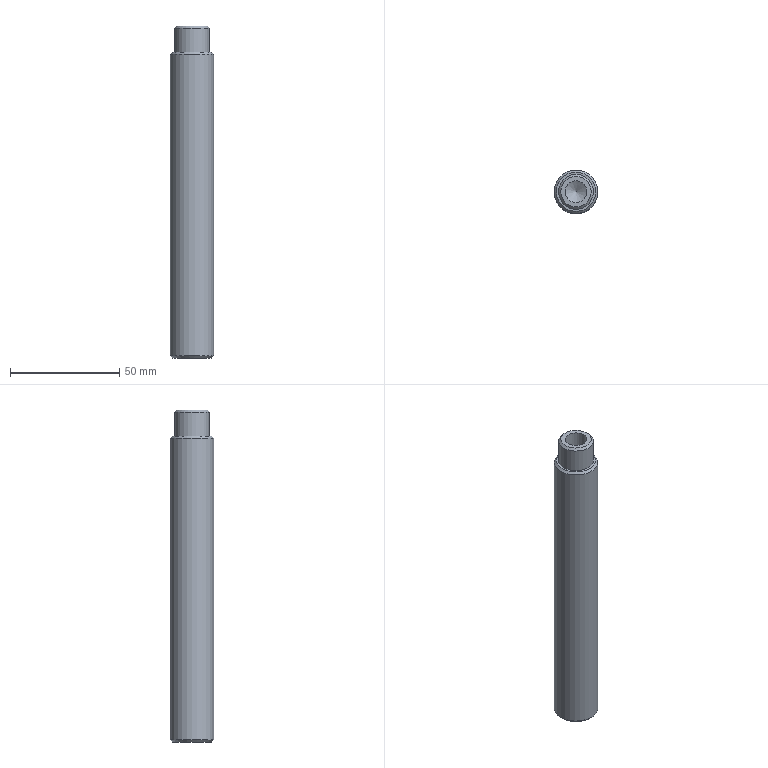Component | NX | STUD | 1 solid | 12 faces | box 20 x 20 x 152 mm | volume 43662 mm3 | cone 5 | cylinder 4 | plane 3 | commonest cylinder face diameters 20 x1 16 x1 6.8 x1 10 x1
STEP:
#1=CARTESIAN_POINT('',(0.,0.,0.));
#2=DIRECTION('',(0.,0.,1.));
#3=DIRECTION('',(1.,0.,0.));
#4=AXIS2_PLACEMENT_3D('',#1,#2,#3);
#5=CARTESIAN_POINT('',(-177.087,0.,160.));
#6=VERTEX_POINT('',#5);
#7=CARTESIAN_POINT('',(-186.087,0.,160.));
#8=DIRECTION('',(0.,0.,1.));
#9=DIRECTION('',(1.,0.,0.));
#10=AXIS2_PLACEMENT_3D('',#7,#8,#9);
#11=CIRCLE('',#10,9.);
#12=CARTESIAN_POINT('',(-186.087,0.,160.));
#13=DIRECTION('',(0.,0.,1.));
#14=DIRECTION('',(1.,0.,0.));
#15=AXIS2_PLACEMENT_3D('',#12,#13,#14);
#16=PLANE('',#15);
#17=CARTESIAN_POINT('',(0.,0.));
#18=DIRECTION('',(1.,0.));
#19=AXIS2_PLACEMENT_2D('',#17,#18);
#20=CIRCLE('',#19,9.);
#21=(GEOMETRIC_REPRESENTATION_CONTEXT(2)PARAMETRIC_REPRESENTATION_CONTEXT()REPRESENTATION_CONTEXT('',''));
#22=DEFINITIONAL_REPRESENTATION('',(#20),#21);
#23=PCURVE('',#16,#22);
#24=CARTESIAN_POINT('',(-186.087,0.,159.));
#25=DIRECTION('',(0.,0.,-1.));
#26=DIRECTION('',(-1.,0.,0.));
#27=AXIS2_PLACEMENT_3D('',#24,#25,#26);
#28=CONICAL_SURFACE('',#27,10.,0.7854);
#29=CARTESIAN_POINT('',(9.425,-1.));
#30=DIRECTION('',(-1.,0.));
#31=VECTOR('',#30,1.);
#32=LINE('',#29,#31);
#33=(GEOMETRIC_REPRESENTATION_CONTEXT(2)PARAMETRIC_REPRESENTATION_CONTEXT()REPRESENTATION_CONTEXT('',''));
#34=DEFINITIONAL_REPRESENTATION('',(#32),#33);
#35=PCURVE('',#28,#34);
#36=SURFACE_CURVE('',#11,(#23,#35),.PCURVE_S1.);
#37=EDGE_CURVE('',#6,#6,#36,.T.);
#38=ORIENTED_EDGE('',*,*,#37,.T.);
#39=EDGE_LOOP('',(#38));
#40=FACE_BOUND('',#39,.T.);
#41=CARTESIAN_POINT('',(-178.087,0.,160.));
#42=VERTEX_POINT('',#41);
#43=CARTESIAN_POINT('',(-186.087,0.,160.));
#44=DIRECTION('',(0.,0.,1.));
#45=DIRECTION('',(1.,0.,0.));
#46=AXIS2_PLACEMENT_3D('',#43,#44,#45);
#47=CIRCLE('',#46,8.);
#48=CARTESIAN_POINT('',(0.,0.));
#49=DIRECTION('',(1.,0.));
#50=AXIS2_PLACEMENT_2D('',#48,#49);
#51=CIRCLE('',#50,8.);
#52=(GEOMETRIC_REPRESENTATION_CONTEXT(2)PARAMETRIC_REPRESENTATION_CONTEXT()REPRESENTATION_CONTEXT('',''));
#53=DEFINITIONAL_REPRESENTATION('',(#51),#52);
#54=PCURVE('',#16,#53);
#55=CARTESIAN_POINT('',(-186.087,0.,172.));
#56=DIRECTION('',(0.,0.,-1.));
#57=DIRECTION('',(-1.,0.,0.));
#58=AXIS2_PLACEMENT_3D('',#55,#56,#57);
#59=CYLINDRICAL_SURFACE('',#58,8.);
#60=CARTESIAN_POINT('',(9.425,12.));
#61=DIRECTION('',(-1.,0.));
#62=VECTOR('',#61,1.);
#63=LINE('',#60,#62);
#64=(GEOMETRIC_REPRESENTATION_CONTEXT(2)PARAMETRIC_REPRESENTATION_CONTEXT()REPRESENTATION_CONTEXT('',''));
#65=DEFINITIONAL_REPRESENTATION('',(#63),#64);
#66=PCURVE('',#59,#65);
#67=SURFACE_CURVE('',#47,(#54,#66),.PCURVE_S1.);
#68=EDGE_CURVE('',#42,#42,#67,.T.);
#69=ORIENTED_EDGE('',*,*,#68,.F.);
#70=EDGE_LOOP('',(#69));
#71=FACE_BOUND('',#70,.T.);
#72=ADVANCED_FACE('',(#40,#71),#16,.T.);
#73=CARTESIAN_POINT('',(-195.087,0.,20.));
#74=VERTEX_POINT('',#73);
#75=CARTESIAN_POINT('',(-186.087,0.,20.));
#76=DIRECTION('',(0.,0.,-1.));
#77=DIRECTION('',(-1.,0.,0.));
#78=AXIS2_PLACEMENT_3D('',#75,#76,#77);
#79=CIRCLE('',#78,9.);
#80=CARTESIAN_POINT('',(-186.087,0.,20.));
#81=DIRECTION('',(0.,0.,-1.));
#82=DIRECTION('',(-1.,0.,0.));
#83=AXIS2_PLACEMENT_3D('',#80,#81,#82);
#84=PLANE('',#83);
#85=CARTESIAN_POINT('',(0.,0.));
#86=DIRECTION('',(1.,0.));
#87=AXIS2_PLACEMENT_2D('',#85,#86);
#88=CIRCLE('',#87,9.);
#89=(GEOMETRIC_REPRESENTATION_CONTEXT(2)PARAMETRIC_REPRESENTATION_CONTEXT()REPRESENTATION_CONTEXT('',''));
#90=DEFINITIONAL_REPRESENTATION('',(#88),#89);
#91=PCURVE('',#84,#90);
#92=CARTESIAN_POINT('',(-186.087,0.,21.));
#93=DIRECTION('',(0.,0.,1.));
#94=DIRECTION('',(1.,0.,0.));
#95=AXIS2_PLACEMENT_3D('',#92,#93,#94);
#96=CONICAL_SURFACE('',#95,10.,0.7854);
#97=CARTESIAN_POINT('',(9.425,-1.));
#98=DIRECTION('',(-1.,0.));
#99=VECTOR('',#98,1.);
#100=LINE('',#97,#99);
#101=(GEOMETRIC_REPRESENTATION_CONTEXT(2)PARAMETRIC_REPRESENTATION_CONTEXT()REPRESENTATION_CONTEXT('',''));
#102=DEFINITIONAL_REPRESENTATION('',(#100),#101);
#103=PCURVE('',#96,#102);
#104=SURFACE_CURVE('',#79,(#91,#103),.PCURVE_S1.);
#105=EDGE_CURVE('',#74,#74,#104,.T.);
#106=ORIENTED_EDGE('',*,*,#105,.T.);
#107=EDGE_LOOP('',(#106));
#108=FACE_BOUND('',#107,.T.);
#109=CARTESIAN_POINT('',(-182.687,0.,20.));
#110=VERTEX_POINT('',#109);
#111=CARTESIAN_POINT('',(-186.087,0.,20.));
#112=DIRECTION('',(0.,0.,1.));
#113=DIRECTION('',(1.,0.,0.));
#114=AXIS2_PLACEMENT_3D('',#111,#112,#113);
#115=CIRCLE('',#114,3.4);
#116=CARTESIAN_POINT('',(-3.4,0.));
#117=CARTESIAN_POINT('',(-3.4,5.889));
#118=CARTESIAN_POINT('',(1.7,2.944));
#119=CARTESIAN_POINT('',(6.8,0.));
#120=CARTESIAN_POINT('',(1.7,-2.944));
#121=CARTESIAN_POINT('',(-3.4,-5.889));
#122=CARTESIAN_POINT('',(-3.4,0.));
#123=(BOUNDED_CURVE()B_SPLINE_CURVE(2,(#116,#117,#118,#119,#120,#121,#122),.UNSPECIFIED.,.T.,.F.)B_SPLINE_CURVE_WITH_KNOTS((1,2,2,2,2,1),(-2.094,0.,2.094,4.189,6.283,8.378),.UNSPECIFIED.)CURVE()GEOMETRIC_REPRESENTATION_ITEM()RATIONAL_B_SPLINE_CURVE((1.,0.5,1.,0.5,1.,0.5,1.))REPRESENTATION_ITEM(''));
#124=(GEOMETRIC_REPRESENTATION_CONTEXT(2)PARAMETRIC_REPRESENTATION_CONTEXT()REPRESENTATION_CONTEXT('',''));
#125=DEFINITIONAL_REPRESENTATION('',(#123),#124);
#126=PCURVE('',#84,#125);
#127=CARTESIAN_POINT('',(-186.087,0.,20.));
#128=DIRECTION('',(0.,0.,1.));
#129=DIRECTION('',(1.,0.,0.));
#130=AXIS2_PLACEMENT_3D('',#127,#128,#129);
#131=CYLINDRICAL_SURFACE('',#130,3.4);
#132=CARTESIAN_POINT('',(0.,0.));
#133=DIRECTION('',(1.,0.));
#134=VECTOR('',#133,1.);
#135=LINE('',#132,#134);
#136=(GEOMETRIC_REPRESENTATION_CONTEXT(2)PARAMETRIC_REPRESENTATION_CONTEXT()REPRESENTATION_CONTEXT('',''));
#137=DEFINITIONAL_REPRESENTATION('',(#135),#136);
#138=PCURVE('',#131,#137);
#139=SURFACE_CURVE('',#115,(#126,#138),.PCURVE_S1.);
#140=EDGE_CURVE('',#110,#110,#139,.T.);
#141=ORIENTED_EDGE('',*,*,#140,.T.);
#142=EDGE_LOOP('',(#141));
#143=FACE_BOUND('',#142,.T.);
#144=ADVANCED_FACE('',(#108,#143),#84,.T.);
#145=CARTESIAN_POINT('',(-176.087,0.,159.));
#146=VERTEX_POINT('',#145);
#147=CARTESIAN_POINT('',(-186.087,0.,159.));
#148=DIRECTION('',(0.,0.,-1.));
#149=DIRECTION('',(1.,0.,0.));
#150=AXIS2_PLACEMENT_3D('',#147,#148,#149);
#151=CIRCLE('',#150,10.);
#152=CARTESIAN_POINT('',(-186.087,0.,20.));
#153=DIRECTION('',(0.,0.,1.));
#154=DIRECTION('',(1.,0.,0.));
#155=AXIS2_PLACEMENT_3D('',#152,#153,#154);
#156=CYLINDRICAL_SURFACE('',#155,10.);
#157=CARTESIAN_POINT('',(6.283,139.));
#158=DIRECTION('',(-1.,0.));
#159=VECTOR('',#158,1.);
#160=LINE('',#157,#159);
#161=(GEOMETRIC_REPRESENTATION_CONTEXT(2)PARAMETRIC_REPRESENTATION_CONTEXT()REPRESENTATION_CONTEXT('',''));
#162=DEFINITIONAL_REPRESENTATION('',(#160),#161);
#163=PCURVE('',#156,#162);
#164=CARTESIAN_POINT('',(3.142,0.));
#165=DIRECTION('',(1.,0.));
#166=VECTOR('',#165,1.);
#167=LINE('',#164,#166);
#168=(GEOMETRIC_REPRESENTATION_CONTEXT(2)PARAMETRIC_REPRESENTATION_CONTEXT()REPRESENTATION_CONTEXT('',''));
#169=DEFINITIONAL_REPRESENTATION('',(#167),#168);
#170=PCURVE('',#28,#169);
#171=SURFACE_CURVE('',#151,(#163,#170),.PCURVE_S1.);
#172=EDGE_CURVE('',#146,#146,#171,.T.);
#173=ORIENTED_EDGE('',*,*,#172,.T.);
#174=CARTESIAN_POINT('',(-176.087,0.,21.));
#175=VERTEX_POINT('',#174);
#176=CARTESIAN_POINT('',(-176.087,0.,21.));
#177=CARTESIAN_POINT('',(-176.087,0.,159.));
#178=B_SPLINE_CURVE_WITH_KNOTS('',1,(#176,#177),.UNSPECIFIED.,.F.,.F.,(2,2),(1.,139.),.PIECEWISE_BEZIER_KNOTS.);
#179=CARTESIAN_POINT('',(0.,0.));
#180=DIRECTION('',(0.,1.));
#181=VECTOR('',#180,1.);
#182=LINE('',#179,#181);
#183=(GEOMETRIC_REPRESENTATION_CONTEXT(2)PARAMETRIC_REPRESENTATION_CONTEXT()REPRESENTATION_CONTEXT('',''));
#184=DEFINITIONAL_REPRESENTATION('',(#182),#183);
#185=PCURVE('',#156,#184);
#186=CARTESIAN_POINT('',(6.283,0.));
#187=DIRECTION('',(0.,1.));
#188=VECTOR('',#187,1.);
#189=LINE('',#186,#188);
#190=(GEOMETRIC_REPRESENTATION_CONTEXT(2)PARAMETRIC_REPRESENTATION_CONTEXT()REPRESENTATION_CONTEXT('',''));
#191=DEFINITIONAL_REPRESENTATION('',(#189),#190);
#192=PCURVE('',#156,#191);
#193=SEAM_CURVE('',#178,(#185,#192),.PCURVE_S1.);
#194=EDGE_CURVE('',#175,#146,#193,.T.);
#195=ORIENTED_EDGE('',*,*,#194,.F.);
#196=CARTESIAN_POINT('',(-196.087,0.,21.));
#197=VERTEX_POINT('',#196);
#198=CARTESIAN_POINT('',(-186.087,0.,21.));
#199=DIRECTION('',(0.,0.,1.));
#200=DIRECTION('',(-1.,0.,0.));
#201=AXIS2_PLACEMENT_3D('',#198,#199,#200);
#202=CIRCLE('',#201,10.);
#203=CARTESIAN_POINT('',(-3.142,1.));
#204=DIRECTION('',(1.,0.));
#205=VECTOR('',#204,1.);
#206=LINE('',#203,#205);
#207=(GEOMETRIC_REPRESENTATION_CONTEXT(2)PARAMETRIC_REPRESENTATION_CONTEXT()REPRESENTATION_CONTEXT('',''));
#208=DEFINITIONAL_REPRESENTATION('',(#206),#207);
#209=PCURVE('',#156,#208);
#210=CARTESIAN_POINT('',(3.142,0.));
#211=DIRECTION('',(1.,0.));
#212=VECTOR('',#211,1.);
#213=LINE('',#210,#212);
#214=(GEOMETRIC_REPRESENTATION_CONTEXT(2)PARAMETRIC_REPRESENTATION_CONTEXT()REPRESENTATION_CONTEXT('',''));
#215=DEFINITIONAL_REPRESENTATION('',(#213),#214);
#216=PCURVE('',#96,#215);
#217=SURFACE_CURVE('',#202,(#209,#216),.PCURVE_S1.);
#218=EDGE_CURVE('',#175,#197,#217,.T.);
#219=ORIENTED_EDGE('',*,*,#218,.T.);
#220=CARTESIAN_POINT('',(-186.087,0.,21.));
#221=DIRECTION('',(0.,0.,1.));
#222=DIRECTION('',(-1.,0.,0.));
#223=AXIS2_PLACEMENT_3D('',#220,#221,#222);
#224=CIRCLE('',#223,10.);
#225=CARTESIAN_POINT('',(3.142,1.));
#226=DIRECTION('',(1.,0.));
#227=VECTOR('',#226,1.);
#228=LINE('',#225,#227);
#229=(GEOMETRIC_REPRESENTATION_CONTEXT(2)PARAMETRIC_REPRESENTATION_CONTEXT()REPRESENTATION_CONTEXT('',''));
#230=DEFINITIONAL_REPRESENTATION('',(#228),#229);
#231=PCURVE('',#156,#230);
#232=CARTESIAN_POINT('',(3.142,0.));
#233=DIRECTION('',(1.,0.));
#234=VECTOR('',#233,1.);
#235=LINE('',#232,#234);
#236=(GEOMETRIC_REPRESENTATION_CONTEXT(2)PARAMETRIC_REPRESENTATION_CONTEXT()REPRESENTATION_CONTEXT('',''));
#237=DEFINITIONAL_REPRESENTATION('',(#235),#236);
#238=PCURVE('',#96,#237);
#239=SURFACE_CURVE('',#224,(#231,#238),.PCURVE_S1.);
#240=EDGE_CURVE('',#197,#175,#239,.T.);
#241=ORIENTED_EDGE('',*,*,#240,.T.);
#242=ORIENTED_EDGE('',*,*,#194,.T.);
#243=EDGE_LOOP('',(#173,#195,#219,#241,#242));
#244=FACE_BOUND('',#243,.T.);
#245=ADVANCED_FACE('',(#244),#156,.T.);
#246=CARTESIAN_POINT('',(-178.087,0.,171.));
#247=VERTEX_POINT('',#246);
#248=CARTESIAN_POINT('',(-186.087,0.,171.));
#249=DIRECTION('',(0.,0.,-1.));
#250=DIRECTION('',(1.,0.,0.));
#251=AXIS2_PLACEMENT_3D('',#248,#249,#250);
#252=CIRCLE('',#251,8.);
#253=CARTESIAN_POINT('',(3.142,1.));
#254=DIRECTION('',(1.,0.));
#255=VECTOR('',#254,1.);
#256=LINE('',#253,#255);
#257=(GEOMETRIC_REPRESENTATION_CONTEXT(2)PARAMETRIC_REPRESENTATION_CONTEXT()REPRESENTATION_CONTEXT('',''));
#258=DEFINITIONAL_REPRESENTATION('',(#256),#257);
#259=PCURVE('',#59,#258);
#260=CARTESIAN_POINT('',(-186.087,0.,172.));
#261=DIRECTION('',(0.,0.,-1.));
#262=DIRECTION('',(-1.,0.,0.));
#263=AXIS2_PLACEMENT_3D('',#260,#261,#262);
#264=CONICAL_SURFACE('',#263,7.,0.7854);
#265=CARTESIAN_POINT('',(3.142,1.));
#266=DIRECTION('',(1.,0.));
#267=VECTOR('',#266,1.);
#268=LINE('',#265,#267);
#269=(GEOMETRIC_REPRESENTATION_CONTEXT(2)PARAMETRIC_REPRESENTATION_CONTEXT()REPRESENTATION_CONTEXT('',''));
#270=DEFINITIONAL_REPRESENTATION('',(#268),#269);
#271=PCURVE('',#264,#270);
#272=SURFACE_CURVE('',#252,(#259,#271),.PCURVE_S1.);
#273=EDGE_CURVE('',#247,#247,#272,.T.);
#274=ORIENTED_EDGE('',*,*,#273,.T.);
#275=CARTESIAN_POINT('',(-178.087,0.,171.));
#276=CARTESIAN_POINT('',(-178.087,0.,160.));
#277=B_SPLINE_CURVE_WITH_KNOTS('',1,(#275,#276),.UNSPECIFIED.,.F.,.F.,(2,2),(1.,12.),.PIECEWISE_BEZIER_KNOTS.);
#278=CARTESIAN_POINT('',(9.425,0.));
#279=DIRECTION('',(0.,1.));
#280=VECTOR('',#279,1.);
#281=LINE('',#278,#280);
#282=(GEOMETRIC_REPRESENTATION_CONTEXT(2)PARAMETRIC_REPRESENTATION_CONTEXT()REPRESENTATION_CONTEXT('',''));
#283=DEFINITIONAL_REPRESENTATION('',(#281),#282);
#284=PCURVE('',#59,#283);
#285=CARTESIAN_POINT('',(3.142,0.));
#286=DIRECTION('',(0.,1.));
#287=VECTOR('',#286,1.);
#288=LINE('',#285,#287);
#289=(GEOMETRIC_REPRESENTATION_CONTEXT(2)PARAMETRIC_REPRESENTATION_CONTEXT()REPRESENTATION_CONTEXT('',''));
#290=DEFINITIONAL_REPRESENTATION('',(#288),#289);
#291=PCURVE('',#59,#290);
#292=SEAM_CURVE('',#277,(#284,#291),.PCURVE_S1.);
#293=EDGE_CURVE('',#247,#42,#292,.T.);
#294=ORIENTED_EDGE('',*,*,#293,.T.);
#295=ORIENTED_EDGE('',*,*,#68,.T.);
#296=ORIENTED_EDGE('',*,*,#293,.F.);
#297=EDGE_LOOP('',(#274,#294,#295,#296));
#298=FACE_BOUND('',#297,.T.);
#299=ADVANCED_FACE('',(#298),#59,.T.);
#300=CARTESIAN_POINT('',(-179.087,0.,172.));
#301=VERTEX_POINT('',#300);
#302=CARTESIAN_POINT('',(-186.087,0.,172.));
#303=DIRECTION('',(0.,0.,1.));
#304=DIRECTION('',(1.,0.,0.));
#305=AXIS2_PLACEMENT_3D('',#302,#303,#304);
#306=CIRCLE('',#305,7.);
#307=CARTESIAN_POINT('',(-186.087,0.,172.));
#308=DIRECTION('',(0.,0.,1.));
#309=DIRECTION('',(1.,0.,0.));
#310=AXIS2_PLACEMENT_3D('',#307,#308,#309);
#311=PLANE('',#310);
#312=CARTESIAN_POINT('',(0.,0.));
#313=DIRECTION('',(1.,0.));
#314=AXIS2_PLACEMENT_2D('',#312,#313);
#315=CIRCLE('',#314,7.);
#316=(GEOMETRIC_REPRESENTATION_CONTEXT(2)PARAMETRIC_REPRESENTATION_CONTEXT()REPRESENTATION_CONTEXT('',''));
#317=DEFINITIONAL_REPRESENTATION('',(#315),#316);
#318=PCURVE('',#311,#317);
#319=CARTESIAN_POINT('',(9.425,0.));
#320=DIRECTION('',(-1.,0.));
#321=VECTOR('',#320,1.);
#322=LINE('',#319,#321);
#323=(GEOMETRIC_REPRESENTATION_CONTEXT(2)PARAMETRIC_REPRESENTATION_CONTEXT()REPRESENTATION_CONTEXT('',''));
#324=DEFINITIONAL_REPRESENTATION('',(#322),#323);
#325=PCURVE('',#264,#324);
#326=SURFACE_CURVE('',#306,(#318,#325),.PCURVE_S1.);
#327=EDGE_CURVE('',#301,#301,#326,.T.);
#328=ORIENTED_EDGE('',*,*,#327,.T.);
#329=EDGE_LOOP('',(#328));
#330=FACE_BOUND('',#329,.T.);
#331=CARTESIAN_POINT('',(-191.087,0.,172.));
#332=VERTEX_POINT('',#331);
#333=CARTESIAN_POINT('',(-186.087,0.,172.));
#334=DIRECTION('',(0.,0.,-1.));
#335=DIRECTION('',(-1.,0.,0.));
#336=AXIS2_PLACEMENT_3D('',#333,#334,#335);
#337=CIRCLE('',#336,5.);
#338=CARTESIAN_POINT('',(-5.,0.));
#339=CARTESIAN_POINT('',(-5.,8.66));
#340=CARTESIAN_POINT('',(2.5,4.33));
#341=CARTESIAN_POINT('',(10.,0.));
#342=CARTESIAN_POINT('',(2.5,-4.33));
#343=CARTESIAN_POINT('',(-5.,-8.66));
#344=CARTESIAN_POINT('',(-5.,0.));
#345=(BOUNDED_CURVE()B_SPLINE_CURVE(2,(#338,#339,#340,#341,#342,#343,#344),.UNSPECIFIED.,.T.,.F.)B_SPLINE_CURVE_WITH_KNOTS((1,2,2,2,2,1),(-2.094,0.,2.094,4.189,6.283,8.378),.UNSPECIFIED.)CURVE()GEOMETRIC_REPRESENTATION_ITEM()RATIONAL_B_SPLINE_CURVE((1.,0.5,1.,0.5,1.,0.5,1.))REPRESENTATION_ITEM(''));
#346=(GEOMETRIC_REPRESENTATION_CONTEXT(2)PARAMETRIC_REPRESENTATION_CONTEXT()REPRESENTATION_CONTEXT('',''));
#347=DEFINITIONAL_REPRESENTATION('',(#345),#346);
#348=PCURVE('',#311,#347);
#349=CARTESIAN_POINT('',(-186.087,0.,172.));
#350=DIRECTION('',(0.,0.,-1.));
#351=DIRECTION('',(-1.,0.,0.));
#352=AXIS2_PLACEMENT_3D('',#349,#350,#351);
#353=CYLINDRICAL_SURFACE('',#352,5.);
#354=CARTESIAN_POINT('',(0.,0.));
#355=DIRECTION('',(1.,0.));
#356=VECTOR('',#355,1.);
#357=LINE('',#354,#356);
#358=(GEOMETRIC_REPRESENTATION_CONTEXT(2)PARAMETRIC_REPRESENTATION_CONTEXT()REPRESENTATION_CONTEXT('',''));
#359=DEFINITIONAL_REPRESENTATION('',(#357),#358);
#360=PCURVE('',#353,#359);
#361=SURFACE_CURVE('',#337,(#348,#360),.PCURVE_S1.);
#362=EDGE_CURVE('',#332,#332,#361,.T.);
#363=ORIENTED_EDGE('',*,*,#362,.T.);
#364=EDGE_LOOP('',(#363));
#365=FACE_BOUND('',#364,.T.);
#366=ADVANCED_FACE('',(#330,#365),#311,.T.);
#367=CARTESIAN_POINT('',(-189.487,0.,36.));
#368=VERTEX_POINT('',#367);
#369=CARTESIAN_POINT('',(-182.687,0.,36.));
#370=VERTEX_POINT('',#369);
#371=CARTESIAN_POINT('',(-186.087,0.,36.));
#372=DIRECTION('',(0.,0.,-1.));
#373=DIRECTION('',(1.,0.,0.));
#374=AXIS2_PLACEMENT_3D('',#371,#372,#373);
#375=CIRCLE('',#374,3.4);
#376=CARTESIAN_POINT('',(-186.087,0.,36.));
#377=DIRECTION('',(0.,0.,-1.));
#378=DIRECTION('',(-1.,0.,0.));
#379=AXIS2_PLACEMENT_3D('',#376,#377,#378);
#380=CONICAL_SURFACE('',#379,3.4,1.03);
#381=CARTESIAN_POINT('',(-3.142,0.));
#382=DIRECTION('',(1.,0.));
#383=VECTOR('',#382,1.);
#384=LINE('',#381,#383);
#385=(GEOMETRIC_REPRESENTATION_CONTEXT(2)PARAMETRIC_REPRESENTATION_CONTEXT()REPRESENTATION_CONTEXT('',''));
#386=DEFINITIONAL_REPRESENTATION('',(#384),#385);
#387=PCURVE('',#380,#386);
#388=CARTESIAN_POINT('',(6.283,16.));
#389=DIRECTION('',(-1.,0.));
#390=VECTOR('',#389,1.);
#391=LINE('',#388,#390);
#392=(GEOMETRIC_REPRESENTATION_CONTEXT(2)PARAMETRIC_REPRESENTATION_CONTEXT()REPRESENTATION_CONTEXT('',''));
#393=DEFINITIONAL_REPRESENTATION('',(#391),#392);
#394=PCURVE('',#131,#393);
#395=SURFACE_CURVE('',#375,(#387,#394),.PCURVE_S1.);
#396=EDGE_CURVE('',#368,#370,#395,.T.);
#397=ORIENTED_EDGE('',*,*,#396,.F.);
#398=CARTESIAN_POINT('',(-186.087,0.,38.043));
#399=VERTEX_POINT('',#398);
#400=CARTESIAN_POINT('',(-186.087,0.,38.043));
#401=CARTESIAN_POINT('',(-189.487,0.,36.));
#402=B_SPLINE_CURVE_WITH_KNOTS('',1,(#400,#401),.UNSPECIFIED.,.F.,.F.,(2,2),(-3.967,0.),.PIECEWISE_BEZIER_KNOTS.);
#403=CARTESIAN_POINT('',(0.,0.));
#404=DIRECTION('',(0.,1.));
#405=VECTOR('',#404,1.);
#406=LINE('',#403,#405);
#407=(GEOMETRIC_REPRESENTATION_CONTEXT(2)PARAMETRIC_REPRESENTATION_CONTEXT()REPRESENTATION_CONTEXT('',''));
#408=DEFINITIONAL_REPRESENTATION('',(#406),#407);
#409=PCURVE('',#380,#408);
#410=CARTESIAN_POINT('',(6.283,0.));
#411=DIRECTION('',(0.,1.));
#412=VECTOR('',#411,1.);
#413=LINE('',#410,#412);
#414=(GEOMETRIC_REPRESENTATION_CONTEXT(2)PARAMETRIC_REPRESENTATION_CONTEXT()REPRESENTATION_CONTEXT('',''));
#415=DEFINITIONAL_REPRESENTATION('',(#413),#414);
#416=PCURVE('',#380,#415);
#417=SEAM_CURVE('',#402,(#409,#416),.PCURVE_S1.);
#418=EDGE_CURVE('',#399,#368,#417,.T.);
#419=ORIENTED_EDGE('',*,*,#418,.F.);
#420=ORIENTED_EDGE('',*,*,#418,.T.);
#421=CARTESIAN_POINT('',(-186.087,0.,36.));
#422=DIRECTION('',(0.,0.,-1.));
#423=DIRECTION('',(1.,0.,0.));
#424=AXIS2_PLACEMENT_3D('',#421,#422,#423);
#425=CIRCLE('',#424,3.4);
#426=CARTESIAN_POINT('',(3.142,0.));
#427=DIRECTION('',(1.,0.));
#428=VECTOR('',#427,1.);
#429=LINE('',#426,#428);
#430=(GEOMETRIC_REPRESENTATION_CONTEXT(2)PARAMETRIC_REPRESENTATION_CONTEXT()REPRESENTATION_CONTEXT('',''));
#431=DEFINITIONAL_REPRESENTATION('',(#429),#430);
#432=PCURVE('',#380,#431);
#433=CARTESIAN_POINT('',(6.283,16.));
#434=DIRECTION('',(-1.,0.));
#435=VECTOR('',#434,1.);
#436=LINE('',#433,#435);
#437=(GEOMETRIC_REPRESENTATION_CONTEXT(2)PARAMETRIC_REPRESENTATION_CONTEXT()REPRESENTATION_CONTEXT('',''));
#438=DEFINITIONAL_REPRESENTATION('',(#436),#437);
#439=PCURVE('',#131,#438);
#440=SURFACE_CURVE('',#425,(#432,#439),.PCURVE_S1.);
#441=EDGE_CURVE('',#370,#368,#440,.T.);
#442=ORIENTED_EDGE('',*,*,#441,.F.);
#443=EDGE_LOOP('',(#397,#419,#420,#442));
#444=FACE_BOUND('',#443,.F.);
#445=ADVANCED_FACE('',(#444),#380,.F.);
#446=ORIENTED_EDGE('',*,*,#396,.T.);
#447=CARTESIAN_POINT('',(-182.687,0.,20.));
#448=CARTESIAN_POINT('',(-182.687,0.,36.));
#449=B_SPLINE_CURVE_WITH_KNOTS('',1,(#447,#448),.UNSPECIFIED.,.F.,.F.,(2,2),(0.,16.),.PIECEWISE_BEZIER_KNOTS.);
#450=CARTESIAN_POINT('',(0.,0.));
#451=DIRECTION('',(0.,1.));
#452=VECTOR('',#451,1.);
#453=LINE('',#450,#452);
#454=(GEOMETRIC_REPRESENTATION_CONTEXT(2)PARAMETRIC_REPRESENTATION_CONTEXT()REPRESENTATION_CONTEXT('',''));
#455=DEFINITIONAL_REPRESENTATION('',(#453),#454);
#456=PCURVE('',#131,#455);
#457=CARTESIAN_POINT('',(6.283,0.));
#458=DIRECTION('',(0.,1.));
#459=VECTOR('',#458,1.);
#460=LINE('',#457,#459);
#461=(GEOMETRIC_REPRESENTATION_CONTEXT(2)PARAMETRIC_REPRESENTATION_CONTEXT()REPRESENTATION_CONTEXT('',''));
#462=DEFINITIONAL_REPRESENTATION('',(#460),#461);
#463=PCURVE('',#131,#462);
#464=SEAM_CURVE('',#449,(#456,#463),.PCURVE_S1.);
#465=EDGE_CURVE('',#110,#370,#464,.T.);
#466=ORIENTED_EDGE('',*,*,#465,.F.);
#467=ORIENTED_EDGE('',*,*,#140,.T.);
#468=ORIENTED_EDGE('',*,*,#465,.T.);
#469=ORIENTED_EDGE('',*,*,#441,.T.);
#470=EDGE_LOOP('',(#446,#466,#467,#468,#469));
#471=FACE_BOUND('',#470,.F.);
#472=ADVANCED_FACE('',(#471),#131,.F.);
#473=CARTESIAN_POINT('',(-181.087,0.,147.));
#474=VERTEX_POINT('',#473);
#475=CARTESIAN_POINT('',(-191.087,0.,147.));
#476=VERTEX_POINT('',#475);
#477=CARTESIAN_POINT('',(-186.087,0.,147.));
#478=DIRECTION('',(0.,0.,1.));
#479=DIRECTION('',(-1.,0.,0.));
#480=AXIS2_PLACEMENT_3D('',#477,#478,#479);
#481=CIRCLE('',#480,5.);
#482=CARTESIAN_POINT('',(-186.087,0.,147.));
#483=DIRECTION('',(0.,0.,1.));
#484=DIRECTION('',(1.,0.,0.));
#485=AXIS2_PLACEMENT_3D('',#482,#483,#484);
#486=CONICAL_SURFACE('',#485,5.,1.03);
#487=CARTESIAN_POINT('',(-3.142,0.));
#488=DIRECTION('',(1.,0.));
#489=VECTOR('',#488,1.);
#490=LINE('',#487,#489);
#491=(GEOMETRIC_REPRESENTATION_CONTEXT(2)PARAMETRIC_REPRESENTATION_CONTEXT()REPRESENTATION_CONTEXT('',''));
#492=DEFINITIONAL_REPRESENTATION('',(#490),#491);
#493=PCURVE('',#486,#492);
#494=CARTESIAN_POINT('',(6.283,25.));
#495=DIRECTION('',(-1.,0.));
#496=VECTOR('',#495,1.);
#497=LINE('',#494,#496);
#498=(GEOMETRIC_REPRESENTATION_CONTEXT(2)PARAMETRIC_REPRESENTATION_CONTEXT()REPRESENTATION_CONTEXT('',''));
#499=DEFINITIONAL_REPRESENTATION('',(#497),#498);
#500=PCURVE('',#353,#499);
#501=SURFACE_CURVE('',#481,(#493,#500),.PCURVE_S1.);
#502=EDGE_CURVE('',#474,#476,#501,.T.);
#503=ORIENTED_EDGE('',*,*,#502,.F.);
#504=CARTESIAN_POINT('',(-186.087,0.,143.996));
#505=VERTEX_POINT('',#504);
#506=CARTESIAN_POINT('',(-186.087,0.,143.996));
#507=CARTESIAN_POINT('',(-181.087,0.,147.));
#508=B_SPLINE_CURVE_WITH_KNOTS('',1,(#506,#507),.UNSPECIFIED.,.F.,.F.,(2,2),(-5.833,0.),.PIECEWISE_BEZIER_KNOTS.);
#509=CARTESIAN_POINT('',(0.,0.));
#510=DIRECTION('',(0.,1.));
#511=VECTOR('',#510,1.);
#512=LINE('',#509,#511);
#513=(GEOMETRIC_REPRESENTATION_CONTEXT(2)PARAMETRIC_REPRESENTATION_CONTEXT()REPRESENTATION_CONTEXT('',''));
#514=DEFINITIONAL_REPRESENTATION('',(#512),#513);
#515=PCURVE('',#486,#514);
#516=CARTESIAN_POINT('',(6.283,0.));
#517=DIRECTION('',(0.,1.));
#518=VECTOR('',#517,1.);
#519=LINE('',#516,#518);
#520=(GEOMETRIC_REPRESENTATION_CONTEXT(2)PARAMETRIC_REPRESENTATION_CONTEXT()REPRESENTATION_CONTEXT('',''));
#521=DEFINITIONAL_REPRESENTATION('',(#519),#520);
#522=PCURVE('',#486,#521);
#523=SEAM_CURVE('',#508,(#515,#522),.PCURVE_S1.);
#524=EDGE_CURVE('',#505,#474,#523,.T.);
#525=ORIENTED_EDGE('',*,*,#524,.F.);
#526=ORIENTED_EDGE('',*,*,#524,.T.);
#527=CARTESIAN_POINT('',(-186.087,0.,147.));
#528=DIRECTION('',(0.,0.,1.));
#529=DIRECTION('',(-1.,0.,0.));
#530=AXIS2_PLACEMENT_3D('',#527,#528,#529);
#531=CIRCLE('',#530,5.);
#532=CARTESIAN_POINT('',(3.142,0.));
#533=DIRECTION('',(1.,0.));
#534=VECTOR('',#533,1.);
#535=LINE('',#532,#534);
#536=(GEOMETRIC_REPRESENTATION_CONTEXT(2)PARAMETRIC_REPRESENTATION_CONTEXT()REPRESENTATION_CONTEXT('',''));
#537=DEFINITIONAL_REPRESENTATION('',(#535),#536);
#538=PCURVE('',#486,#537);
#539=CARTESIAN_POINT('',(6.283,25.));
#540=DIRECTION('',(-1.,0.));
#541=VECTOR('',#540,1.);
#542=LINE('',#539,#541);
#543=(GEOMETRIC_REPRESENTATION_CONTEXT(2)PARAMETRIC_REPRESENTATION_CONTEXT()REPRESENTATION_CONTEXT('',''));
#544=DEFINITIONAL_REPRESENTATION('',(#542),#543);
#545=PCURVE('',#353,#544);
#546=SURFACE_CURVE('',#531,(#538,#545),.PCURVE_S1.);
#547=EDGE_CURVE('',#476,#474,#546,.T.);
#548=ORIENTED_EDGE('',*,*,#547,.F.);
#549=EDGE_LOOP('',(#503,#525,#526,#548));
#550=FACE_BOUND('',#549,.F.);
#551=ADVANCED_FACE('',(#550),#486,.F.);
#552=ORIENTED_EDGE('',*,*,#502,.T.);
#553=CARTESIAN_POINT('',(-191.087,0.,172.));
#554=CARTESIAN_POINT('',(-191.087,0.,147.));
#555=B_SPLINE_CURVE_WITH_KNOTS('',1,(#553,#554),.UNSPECIFIED.,.F.,.F.,(2,2),(0.,25.),.PIECEWISE_BEZIER_KNOTS.);
#556=CARTESIAN_POINT('',(0.,0.));
#557=DIRECTION('',(0.,1.));
#558=VECTOR('',#557,1.);
#559=LINE('',#556,#558);
#560=(GEOMETRIC_REPRESENTATION_CONTEXT(2)PARAMETRIC_REPRESENTATION_CONTEXT()REPRESENTATION_CONTEXT('',''));
#561=DEFINITIONAL_REPRESENTATION('',(#559),#560);
#562=PCURVE('',#353,#561);
#563=CARTESIAN_POINT('',(6.283,0.));
#564=DIRECTION('',(0.,1.));
#565=VECTOR('',#564,1.);
#566=LINE('',#563,#565);
#567=(GEOMETRIC_REPRESENTATION_CONTEXT(2)PARAMETRIC_REPRESENTATION_CONTEXT()REPRESENTATION_CONTEXT('',''));
#568=DEFINITIONAL_REPRESENTATION('',(#566),#567);
#569=PCURVE('',#353,#568);
#570=SEAM_CURVE('',#555,(#562,#569),.PCURVE_S1.);
#571=EDGE_CURVE('',#332,#476,#570,.T.);
#572=ORIENTED_EDGE('',*,*,#571,.F.);
#573=ORIENTED_EDGE('',*,*,#362,.T.);
#574=ORIENTED_EDGE('',*,*,#571,.T.);
#575=ORIENTED_EDGE('',*,*,#547,.T.);
#576=EDGE_LOOP('',(#552,#572,#573,#574,#575));
#577=FACE_BOUND('',#576,.F.);
#578=ADVANCED_FACE('',(#577),#353,.F.);
#579=ORIENTED_EDGE('',*,*,#273,.F.);
#580=CARTESIAN_POINT('',(-179.087,0.,172.));
#581=CARTESIAN_POINT('',(-178.087,0.,171.));
#582=B_SPLINE_CURVE_WITH_KNOTS('',1,(#580,#581),.UNSPECIFIED.,.F.,.F.,(2,2),(0.,1.414),.PIECEWISE_BEZIER_KNOTS.);
#583=CARTESIAN_POINT('',(3.142,0.));
#584=DIRECTION('',(0.,1.));
#585=VECTOR('',#584,1.);
#586=LINE('',#583,#585);
#587=(GEOMETRIC_REPRESENTATION_CONTEXT(2)PARAMETRIC_REPRESENTATION_CONTEXT()REPRESENTATION_CONTEXT('',''));
#588=DEFINITIONAL_REPRESENTATION('',(#586),#587);
#589=PCURVE('',#264,#588);
#590=CARTESIAN_POINT('',(9.425,0.));
#591=DIRECTION('',(0.,1.));
#592=VECTOR('',#591,1.);
#593=LINE('',#590,#592);
#594=(GEOMETRIC_REPRESENTATION_CONTEXT(2)PARAMETRIC_REPRESENTATION_CONTEXT()REPRESENTATION_CONTEXT('',''));
#595=DEFINITIONAL_REPRESENTATION('',(#593),#594);
#596=PCURVE('',#264,#595);
#597=SEAM_CURVE('',#582,(#589,#596),.PCURVE_S1.);
#598=EDGE_CURVE('',#301,#247,#597,.T.);
#599=ORIENTED_EDGE('',*,*,#598,.F.);
#600=ORIENTED_EDGE('',*,*,#327,.F.);
#601=ORIENTED_EDGE('',*,*,#598,.T.);
#602=EDGE_LOOP('',(#579,#599,#600,#601));
#603=FACE_BOUND('',#602,.T.);
#604=ADVANCED_FACE('',(#603),#264,.T.);
#605=ORIENTED_EDGE('',*,*,#37,.F.);
#606=CARTESIAN_POINT('',(-177.087,0.,160.));
#607=CARTESIAN_POINT('',(-176.087,0.,159.));
#608=B_SPLINE_CURVE_WITH_KNOTS('',1,(#606,#607),.UNSPECIFIED.,.F.,.F.,(2,2),(-1.414,0.),.PIECEWISE_BEZIER_KNOTS.);
#609=CARTESIAN_POINT('',(9.425,0.));
#610=DIRECTION('',(0.,1.));
#611=VECTOR('',#610,1.);
#612=LINE('',#609,#611);
#613=(GEOMETRIC_REPRESENTATION_CONTEXT(2)PARAMETRIC_REPRESENTATION_CONTEXT()REPRESENTATION_CONTEXT('',''));
#614=DEFINITIONAL_REPRESENTATION('',(#612),#613);
#615=PCURVE('',#28,#614);
#616=CARTESIAN_POINT('',(3.142,0.));
#617=DIRECTION('',(0.,1.));
#618=VECTOR('',#617,1.);
#619=LINE('',#616,#618);
#620=(GEOMETRIC_REPRESENTATION_CONTEXT(2)PARAMETRIC_REPRESENTATION_CONTEXT()REPRESENTATION_CONTEXT('',''));
#621=DEFINITIONAL_REPRESENTATION('',(#619),#620);
#622=PCURVE('',#28,#621);
#623=SEAM_CURVE('',#608,(#615,#622),.PCURVE_S1.);
#624=EDGE_CURVE('',#6,#146,#623,.T.);
#625=ORIENTED_EDGE('',*,*,#624,.T.);
#626=ORIENTED_EDGE('',*,*,#172,.F.);
#627=ORIENTED_EDGE('',*,*,#624,.F.);
#628=EDGE_LOOP('',(#605,#625,#626,#627));
#629=FACE_BOUND('',#628,.T.);
#630=ADVANCED_FACE('',(#629),#28,.T.);
#631=ORIENTED_EDGE('',*,*,#105,.F.);
#632=CARTESIAN_POINT('',(-195.087,0.,20.));
#633=CARTESIAN_POINT('',(-196.087,0.,21.));
#634=B_SPLINE_CURVE_WITH_KNOTS('',1,(#632,#633),.UNSPECIFIED.,.F.,.F.,(2,2),(-1.414,0.),.PIECEWISE_BEZIER_KNOTS.);
#635=CARTESIAN_POINT('',(9.425,0.));
#636=DIRECTION('',(0.,1.));
#637=VECTOR('',#636,1.);
#638=LINE('',#635,#637);
#639=(GEOMETRIC_REPRESENTATION_CONTEXT(2)PARAMETRIC_REPRESENTATION_CONTEXT()REPRESENTATION_CONTEXT('',''));
#640=DEFINITIONAL_REPRESENTATION('',(#638),#639);
#641=PCURVE('',#96,#640);
#642=CARTESIAN_POINT('',(3.142,0.));
#643=DIRECTION('',(0.,1.));
#644=VECTOR('',#643,1.);
#645=LINE('',#642,#644);
#646=(GEOMETRIC_REPRESENTATION_CONTEXT(2)PARAMETRIC_REPRESENTATION_CONTEXT()REPRESENTATION_CONTEXT('',''));
#647=DEFINITIONAL_REPRESENTATION('',(#645),#646);
#648=PCURVE('',#96,#647);
#649=SEAM_CURVE('',#634,(#641,#648),.PCURVE_S1.);
#650=EDGE_CURVE('',#74,#197,#649,.T.);
#651=ORIENTED_EDGE('',*,*,#650,.T.);
#652=ORIENTED_EDGE('',*,*,#218,.F.);
#653=ORIENTED_EDGE('',*,*,#240,.F.);
#654=ORIENTED_EDGE('',*,*,#650,.F.);
#655=EDGE_LOOP('',(#631,#651,#652,#653,#654));
#656=FACE_BOUND('',#655,.T.);
#657=ADVANCED_FACE('',(#656),#96,.T.);
#658=CLOSED_SHELL('',(#72,#144,#245,#299,#366,#445,#472,#551,#578,#604,#630,#657));
#659=MANIFOLD_SOLID_BREP('',#658);
#660=(LENGTH_UNIT()NAMED_UNIT(*)SI_UNIT(.MILLI.,.METRE.));
#661=UNCERTAINTY_MEASURE_WITH_UNIT(LENGTH_MEASURE(0.00001),#660,'','');
#662=(NAMED_UNIT(*)PLANE_ANGLE_UNIT()SI_UNIT($,.RADIAN.));
#663=(NAMED_UNIT(*)SI_UNIT($,.STERADIAN.)SOLID_ANGLE_UNIT());
#664=(GEOMETRIC_REPRESENTATION_CONTEXT(3)GLOBAL_UNCERTAINTY_ASSIGNED_CONTEXT((#661))GLOBAL_UNIT_ASSIGNED_CONTEXT((#660,#662,#663))REPRESENTATION_CONTEXT('',''));
#665=ADVANCED_BREP_SHAPE_REPRESENTATION('',(#4,#659),#664);